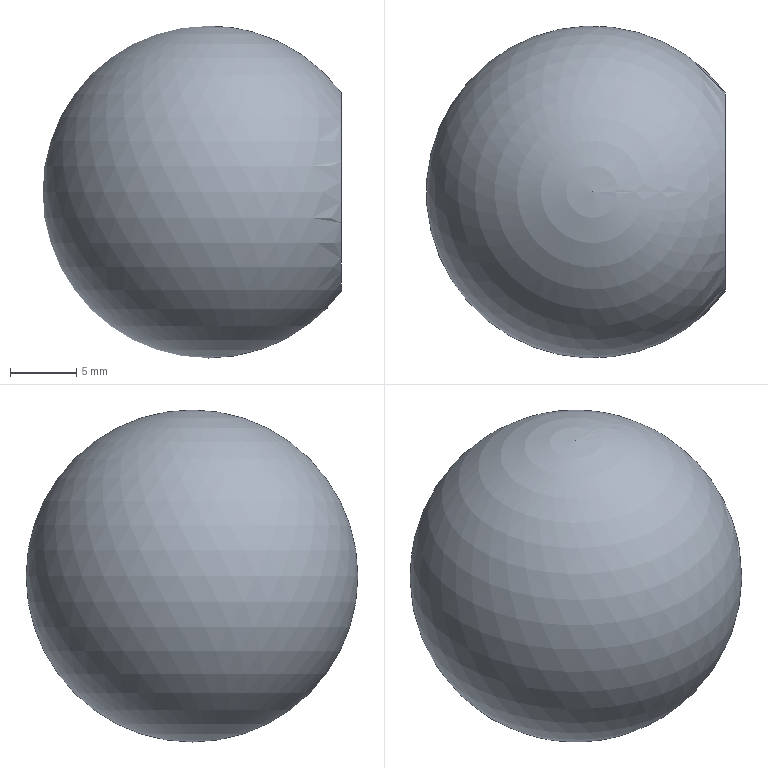Component | NX | HANDLE_1_2 | 1 solid | 4 faces | box 22.5 x 25 x 25 mm | volume 7108 mm3 | plane 1 | sphere 1 | cone 1 | cylinder 1 | commonest cylinder face diameters 8 x1
STEP:
#1=CARTESIAN_POINT('',(0.,0.,0.));
#2=DIRECTION('',(0.,0.,1.));
#3=DIRECTION('',(1.,0.,0.));
#4=AXIS2_PLACEMENT_3D('',#1,#2,#3);
#5=CARTESIAN_POINT('',(-80.,-140.,-185.));
#6=VERTEX_POINT('',#5);
#7=CARTESIAN_POINT('',(-80.,-140.,-189.));
#8=DIRECTION('',(-1.,0.,0.));
#9=DIRECTION('',(0.,0.,1.));
#10=AXIS2_PLACEMENT_3D('',#7,#8,#9);
#11=CIRCLE('',#10,4.);
#12=CARTESIAN_POINT('',(-80.,-140.,-189.));
#13=DIRECTION('',(1.,0.,0.));
#14=DIRECTION('',(0.,0.,-1.));
#15=AXIS2_PLACEMENT_3D('',#12,#13,#14);
#16=PLANE('',#15);
#17=CARTESIAN_POINT('',(-4.,0.));
#18=CARTESIAN_POINT('',(-4.,6.928));
#19=CARTESIAN_POINT('',(2.,3.464));
#20=CARTESIAN_POINT('',(8.,0.));
#21=CARTESIAN_POINT('',(2.,-3.464));
#22=CARTESIAN_POINT('',(-4.,-6.928));
#23=CARTESIAN_POINT('',(-4.,0.));
#24=(BOUNDED_CURVE()B_SPLINE_CURVE(2,(#17,#18,#19,#20,#21,#22,#23),.UNSPECIFIED.,.T.,.F.)B_SPLINE_CURVE_WITH_KNOTS((1,2,2,2,2,1),(-2.094,0.,2.094,4.189,6.283,8.378),.UNSPECIFIED.)CURVE()GEOMETRIC_REPRESENTATION_ITEM()RATIONAL_B_SPLINE_CURVE((1.,0.5,1.,0.5,1.,0.5,1.))REPRESENTATION_ITEM(''));
#25=(GEOMETRIC_REPRESENTATION_CONTEXT(2)PARAMETRIC_REPRESENTATION_CONTEXT()REPRESENTATION_CONTEXT('',''));
#26=DEFINITIONAL_REPRESENTATION('',(#24),#25);
#27=PCURVE('',#16,#26);
#28=CARTESIAN_POINT('',(-80.,-140.,-189.));
#29=DIRECTION('',(-1.,0.,0.));
#30=DIRECTION('',(0.,0.,1.));
#31=AXIS2_PLACEMENT_3D('',#28,#29,#30);
#32=CYLINDRICAL_SURFACE('',#31,4.);
#33=CARTESIAN_POINT('',(0.,0.));
#34=DIRECTION('',(1.,0.));
#35=VECTOR('',#34,1.);
#36=LINE('',#33,#35);
#37=(GEOMETRIC_REPRESENTATION_CONTEXT(2)PARAMETRIC_REPRESENTATION_CONTEXT()REPRESENTATION_CONTEXT('',''));
#38=DEFINITIONAL_REPRESENTATION('',(#36),#37);
#39=PCURVE('',#32,#38);
#40=SURFACE_CURVE('',#11,(#27,#39),.PCURVE_S1.);
#41=EDGE_CURVE('',#6,#6,#40,.T.);
#42=ORIENTED_EDGE('',*,*,#41,.T.);
#43=EDGE_LOOP('',(#42));
#44=FACE_BOUND('',#43,.T.);
#45=CARTESIAN_POINT('',(-80.,-140.,-196.5));
#46=VERTEX_POINT('',#45);
#47=CARTESIAN_POINT('',(-80.,-140.,-189.));
#48=DIRECTION('',(-1.,0.,0.));
#49=DIRECTION('',(0.,0.,-1.));
#50=AXIS2_PLACEMENT_3D('',#47,#48,#49);
#51=CIRCLE('',#50,7.5);
#52=CARTESIAN_POINT('',(7.5,0.));
#53=CARTESIAN_POINT('',(7.5,-12.99));
#54=CARTESIAN_POINT('',(-3.75,-6.495));
#55=CARTESIAN_POINT('',(-15.,-0.));
#56=CARTESIAN_POINT('',(-3.75,6.495));
#57=CARTESIAN_POINT('',(7.5,12.99));
#58=CARTESIAN_POINT('',(7.5,0.));
#59=(BOUNDED_CURVE()B_SPLINE_CURVE(2,(#52,#53,#54,#55,#56,#57,#58),.UNSPECIFIED.,.T.,.F.)B_SPLINE_CURVE_WITH_KNOTS((1,2,2,2,2,1),(-2.094,0.,2.094,4.189,6.283,8.378),.UNSPECIFIED.)CURVE()GEOMETRIC_REPRESENTATION_ITEM()RATIONAL_B_SPLINE_CURVE((1.,0.5,1.,0.5,1.,0.5,1.))REPRESENTATION_ITEM(''));
#60=(GEOMETRIC_REPRESENTATION_CONTEXT(2)PARAMETRIC_REPRESENTATION_CONTEXT()REPRESENTATION_CONTEXT('',''));
#61=DEFINITIONAL_REPRESENTATION('',(#59),#60);
#62=PCURVE('',#16,#61);
#63=CARTESIAN_POINT('',(-90.,-140.,-189.));
#64=DIRECTION('',(0.,0.,1.));
#65=DIRECTION('',(1.,0.,0.));
#66=AXIS2_PLACEMENT_3D('',#63,#64,#65);
#67=SPHERICAL_SURFACE('',#66,12.5);
#68=CARTESIAN_POINT('',(6.283,-0.6435));
#69=CARTESIAN_POINT('',(6.21,-0.644));
#70=CARTESIAN_POINT('',(6.07,-0.6225));
#71=CARTESIAN_POINT('',(5.89,-0.536));
#72=CARTESIAN_POINT('',(5.76,-0.4081));
#73=CARTESIAN_POINT('',(5.677,-0.2543));
#74=CARTESIAN_POINT('',(5.638,-0.08623));
#75=CARTESIAN_POINT('',(5.638,0.08623));
#76=CARTESIAN_POINT('',(5.677,0.2543));
#77=CARTESIAN_POINT('',(5.76,0.4082));
#78=CARTESIAN_POINT('',(5.89,0.5359));
#79=CARTESIAN_POINT('',(6.069,0.6227));
#80=CARTESIAN_POINT('',(6.283,0.6539));
#81=CARTESIAN_POINT('',(6.497,0.6227));
#82=CARTESIAN_POINT('',(6.677,0.5359));
#83=CARTESIAN_POINT('',(6.807,0.4082));
#84=CARTESIAN_POINT('',(6.889,0.2543));
#85=CARTESIAN_POINT('',(6.928,0.08623));
#86=CARTESIAN_POINT('',(6.928,-0.08623));
#87=CARTESIAN_POINT('',(6.889,-0.2543));
#88=CARTESIAN_POINT('',(6.807,-0.4081));
#89=CARTESIAN_POINT('',(6.677,-0.536));
#90=CARTESIAN_POINT('',(6.496,-0.6225));
#91=CARTESIAN_POINT('',(6.356,-0.644));
#92=CARTESIAN_POINT('',(6.283,-0.6435));
#93=B_SPLINE_CURVE_WITH_KNOTS('',3,(#68,#69,#70,#71,#72,#73,#74,#75,#76,#77,#78,#79,#80,#81,#82,#83,#84,#85,#86,#87,#88,#89,#90,#91,#92),.UNSPECIFIED.,.T.,.F.,(4,1,1,1,1,1,1,1,1,1,1,1,1,1,1,1,1,1,1,1,1,1,4),(0.,0.2856,0.5712,0.8568,1.142,1.428,1.714,1.999,2.285,2.57,2.856,3.142,3.427,3.713,3.998,4.284,4.57,4.855,5.141,5.426,5.712,5.998,6.283),.QUASI_UNIFORM_KNOTS.);
#94=(GEOMETRIC_REPRESENTATION_CONTEXT(2)PARAMETRIC_REPRESENTATION_CONTEXT()REPRESENTATION_CONTEXT('',''));
#95=DEFINITIONAL_REPRESENTATION('',(#93),#94);
#96=PCURVE('',#67,#95);
#97=SURFACE_CURVE('',#51,(#62,#96),.PCURVE_S1.);
#98=EDGE_CURVE('',#46,#46,#97,.T.);
#99=ORIENTED_EDGE('',*,*,#98,.F.);
#100=EDGE_LOOP('',(#99));
#101=FACE_BOUND('',#100,.T.);
#102=ADVANCED_FACE('',(#44,#101),#16,.T.);
#103=ORIENTED_EDGE('',*,*,#98,.T.);
#104=EDGE_LOOP('',(#103));
#105=FACE_BOUND('',#104,.T.);
#106=CARTESIAN_POINT('',(-90.,-140.,-201.5));
#107=VERTEX_POINT('',#106);
#108=VERTEX_LOOP('',#107);
#109=FACE_BOUND('',#108,.T.);
#110=ADVANCED_FACE('',(#105,#109),#67,.T.);
#111=CARTESIAN_POINT('',(-96.,-140.,-193.));
#112=VERTEX_POINT('',#111);
#113=CARTESIAN_POINT('',(-96.,-140.,-185.));
#114=VERTEX_POINT('',#113);
#115=CARTESIAN_POINT('',(-96.,-140.,-189.));
#116=DIRECTION('',(1.,0.,0.));
#117=DIRECTION('',(0.,0.,1.));
#118=AXIS2_PLACEMENT_3D('',#115,#116,#117);
#119=CIRCLE('',#118,4.);
#120=CARTESIAN_POINT('',(-96.,-140.,-189.));
#121=DIRECTION('',(1.,0.,0.));
#122=DIRECTION('',(0.,0.,-1.));
#123=AXIS2_PLACEMENT_3D('',#120,#121,#122);
#124=CONICAL_SURFACE('',#123,4.,1.03);
#125=CARTESIAN_POINT('',(-3.142,0.));
#126=DIRECTION('',(1.,0.));
#127=VECTOR('',#126,1.);
#128=LINE('',#125,#127);
#129=(GEOMETRIC_REPRESENTATION_CONTEXT(2)PARAMETRIC_REPRESENTATION_CONTEXT()REPRESENTATION_CONTEXT('',''));
#130=DEFINITIONAL_REPRESENTATION('',(#128),#129);
#131=PCURVE('',#124,#130);
#132=CARTESIAN_POINT('',(6.283,16.));
#133=DIRECTION('',(-1.,0.));
#134=VECTOR('',#133,1.);
#135=LINE('',#132,#134);
#136=(GEOMETRIC_REPRESENTATION_CONTEXT(2)PARAMETRIC_REPRESENTATION_CONTEXT()REPRESENTATION_CONTEXT('',''));
#137=DEFINITIONAL_REPRESENTATION('',(#135),#136);
#138=PCURVE('',#32,#137);
#139=SURFACE_CURVE('',#119,(#131,#138),.PCURVE_S1.);
#140=EDGE_CURVE('',#112,#114,#139,.T.);
#141=ORIENTED_EDGE('',*,*,#140,.F.);
#142=CARTESIAN_POINT('',(-98.403,-140.,-189.));
#143=VERTEX_POINT('',#142);
#144=CARTESIAN_POINT('',(-98.403,-140.,-189.));
#145=CARTESIAN_POINT('',(-96.,-140.,-193.));
#146=B_SPLINE_CURVE_WITH_KNOTS('',1,(#144,#145),.UNSPECIFIED.,.F.,.F.,(2,2),(-4.667,0.),.PIECEWISE_BEZIER_KNOTS.);
#147=CARTESIAN_POINT('',(0.,0.));
#148=DIRECTION('',(0.,1.));
#149=VECTOR('',#148,1.);
#150=LINE('',#147,#149);
#151=(GEOMETRIC_REPRESENTATION_CONTEXT(2)PARAMETRIC_REPRESENTATION_CONTEXT()REPRESENTATION_CONTEXT('',''));
#152=DEFINITIONAL_REPRESENTATION('',(#150),#151);
#153=PCURVE('',#124,#152);
#154=CARTESIAN_POINT('',(6.283,0.));
#155=DIRECTION('',(0.,1.));
#156=VECTOR('',#155,1.);
#157=LINE('',#154,#156);
#158=(GEOMETRIC_REPRESENTATION_CONTEXT(2)PARAMETRIC_REPRESENTATION_CONTEXT()REPRESENTATION_CONTEXT('',''));
#159=DEFINITIONAL_REPRESENTATION('',(#157),#158);
#160=PCURVE('',#124,#159);
#161=SEAM_CURVE('',#146,(#153,#160),.PCURVE_S1.);
#162=EDGE_CURVE('',#143,#112,#161,.T.);
#163=ORIENTED_EDGE('',*,*,#162,.F.);
#164=ORIENTED_EDGE('',*,*,#162,.T.);
#165=CARTESIAN_POINT('',(-96.,-140.,-189.));
#166=DIRECTION('',(1.,0.,0.));
#167=DIRECTION('',(0.,0.,1.));
#168=AXIS2_PLACEMENT_3D('',#165,#166,#167);
#169=CIRCLE('',#168,4.);
#170=CARTESIAN_POINT('',(3.142,0.));
#171=DIRECTION('',(1.,0.));
#172=VECTOR('',#171,1.);
#173=LINE('',#170,#172);
#174=(GEOMETRIC_REPRESENTATION_CONTEXT(2)PARAMETRIC_REPRESENTATION_CONTEXT()REPRESENTATION_CONTEXT('',''));
#175=DEFINITIONAL_REPRESENTATION('',(#173),#174);
#176=PCURVE('',#124,#175);
#177=CARTESIAN_POINT('',(6.283,16.));
#178=DIRECTION('',(-1.,0.));
#179=VECTOR('',#178,1.);
#180=LINE('',#177,#179);
#181=(GEOMETRIC_REPRESENTATION_CONTEXT(2)PARAMETRIC_REPRESENTATION_CONTEXT()REPRESENTATION_CONTEXT('',''));
#182=DEFINITIONAL_REPRESENTATION('',(#180),#181);
#183=PCURVE('',#32,#182);
#184=SURFACE_CURVE('',#169,(#176,#183),.PCURVE_S1.);
#185=EDGE_CURVE('',#114,#112,#184,.T.);
#186=ORIENTED_EDGE('',*,*,#185,.F.);
#187=EDGE_LOOP('',(#141,#163,#164,#186));
#188=FACE_BOUND('',#187,.F.);
#189=ADVANCED_FACE('',(#188),#124,.F.);
#190=ORIENTED_EDGE('',*,*,#140,.T.);
#191=CARTESIAN_POINT('',(-80.,-140.,-185.));
#192=CARTESIAN_POINT('',(-96.,-140.,-185.));
#193=B_SPLINE_CURVE_WITH_KNOTS('',1,(#191,#192),.UNSPECIFIED.,.F.,.F.,(2,2),(0.,16.),.PIECEWISE_BEZIER_KNOTS.);
#194=CARTESIAN_POINT('',(0.,0.));
#195=DIRECTION('',(0.,1.));
#196=VECTOR('',#195,1.);
#197=LINE('',#194,#196);
#198=(GEOMETRIC_REPRESENTATION_CONTEXT(2)PARAMETRIC_REPRESENTATION_CONTEXT()REPRESENTATION_CONTEXT('',''));
#199=DEFINITIONAL_REPRESENTATION('',(#197),#198);
#200=PCURVE('',#32,#199);
#201=CARTESIAN_POINT('',(6.283,0.));
#202=DIRECTION('',(0.,1.));
#203=VECTOR('',#202,1.);
#204=LINE('',#201,#203);
#205=(GEOMETRIC_REPRESENTATION_CONTEXT(2)PARAMETRIC_REPRESENTATION_CONTEXT()REPRESENTATION_CONTEXT('',''));
#206=DEFINITIONAL_REPRESENTATION('',(#204),#205);
#207=PCURVE('',#32,#206);
#208=SEAM_CURVE('',#193,(#200,#207),.PCURVE_S1.);
#209=EDGE_CURVE('',#6,#114,#208,.T.);
#210=ORIENTED_EDGE('',*,*,#209,.F.);
#211=ORIENTED_EDGE('',*,*,#41,.T.);
#212=ORIENTED_EDGE('',*,*,#209,.T.);
#213=ORIENTED_EDGE('',*,*,#185,.T.);
#214=EDGE_LOOP('',(#190,#210,#211,#212,#213));
#215=FACE_BOUND('',#214,.F.);
#216=ADVANCED_FACE('',(#215),#32,.F.);
#217=CLOSED_SHELL('',(#102,#110,#189,#216));
#218=MANIFOLD_SOLID_BREP('',#217);
#219=(LENGTH_UNIT()NAMED_UNIT(*)SI_UNIT(.MILLI.,.METRE.));
#220=UNCERTAINTY_MEASURE_WITH_UNIT(LENGTH_MEASURE(0.000005),#219,'','');
#221=(NAMED_UNIT(*)PLANE_ANGLE_UNIT()SI_UNIT($,.RADIAN.));
#222=(NAMED_UNIT(*)SI_UNIT($,.STERADIAN.)SOLID_ANGLE_UNIT());
#223=(GEOMETRIC_REPRESENTATION_CONTEXT(3)GLOBAL_UNCERTAINTY_ASSIGNED_CONTEXT((#220))GLOBAL_UNIT_ASSIGNED_CONTEXT((#219,#221,#222))REPRESENTATION_CONTEXT('',''));
#224=ADVANCED_BREP_SHAPE_REPRESENTATION('',(#4,#218),#223);